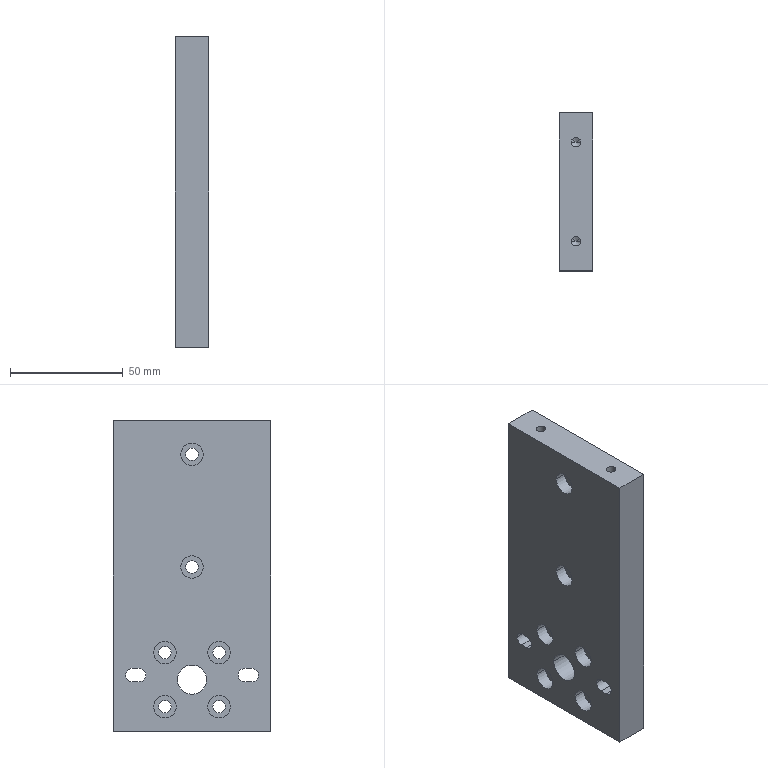Component | SolidWorks | OuterBagSealingSupportPlate-1 | 1 solid | 56 faces | box 15 x 70 x 138 mm | volume 137253 mm3 | cylinder 36 | plane 16 | cone 4 | commonest cylinder face diameters 10 x12 5.5 x12 6 x6 4.2 x4 13 x2
build123d program:
from build123d import *

# Parameters (mm, degrees)
SKETCH1_W                                       = 70
SKETCH1_H                                       = 138
SKETCH1_R                                       = 6.5
BOSS_EXTRUDE1_DEPTH                             = 7.5
M5_HEX_SOCKET_HEAD_CAP_SCREW_CBORE1_D           = 5.5
M5_HEX_SOCKET_HEAD_CAP_SCREW_CBORE1_CBORE_D     = 10
M5_HEX_SOCKET_HEAD_CAP_SCREW_CBORE1_CBORE_DEPTH = 5.4
M5_HEX_SOCKET_HEAD_CAP_SCREW_CBORE2_D           = 5.5
M5_HEX_SOCKET_HEAD_CAP_SCREW_CBORE2_CBORE_D     = 10
M5_HEX_SOCKET_HEAD_CAP_SCREW_CBORE2_CBORE_DEPTH = 5.4
CUT_EXTRUDE1_DEPTH                              = 15
M5_TAPPED_HOLE1_D                               = 4.2
M5_TAPPED_HOLE1_DEPTH                           = 12.4
M5_TAPPED_HOLE1_TIP                             = 1.212


with BuildPart() as part:
    # Sketch1 → Boss-Extrude1 (new, symmetric)
    with BuildSketch(Plane.XY):
        with Locations((35, 69)):
            Rectangle(SKETCH1_W, SKETCH1_H)
        with Locations((35, 115)):
            Circle(SKETCH1_R, mode=Mode.SUBTRACT)
    extrude(amount=BOSS_EXTRUDE1_DEPTH, both=True)

    # M5 Hex Socket Head Cap Screw CBORE1 (through all)
    with Locations(Plane(origin=(23, 127, 7.5), x_dir=(1, 0, 0), z_dir=(0, 0, 1))):
        with Locations((0, 0), (24, 0), (24, -24), (0, -24)):
            CounterBoreHole(M5_HEX_SOCKET_HEAD_CAP_SCREW_CBORE1_D / 2, M5_HEX_SOCKET_HEAD_CAP_SCREW_CBORE1_CBORE_D / 2, M5_HEX_SOCKET_HEAD_CAP_SCREW_CBORE1_CBORE_DEPTH)

    # M5 Hex Socket Head Cap Screw CBORE2 (through all)
    with Locations(Plane(origin=(35, 65, 7.5), x_dir=(1, 0, 0), z_dir=(0, 0, 1))):
        with Locations((0, 0), (0, -50)):
            CounterBoreHole(M5_HEX_SOCKET_HEAD_CAP_SCREW_CBORE2_D / 2, M5_HEX_SOCKET_HEAD_CAP_SCREW_CBORE2_CBORE_D / 2, M5_HEX_SOCKET_HEAD_CAP_SCREW_CBORE2_CBORE_DEPTH)

    # Sketch4 → Cut-Extrude1 (cut)
    with BuildSketch(Plane.XY.offset(7.5)):
        with BuildLine():
            Line((8.5, 116), (11.5, 116))
            ThreePointArc((11.5, 116), (14.5, 113), (11.5, 110))
            Line((11.5, 110), (8.5, 110))
            ThreePointArc((8.5, 110), (5.5, 113), (8.5, 116))
        make_face()
        with BuildLine():
            Line((58.5, 116), (61.5, 116))
            ThreePointArc((61.5, 116), (64.5, 113), (61.5, 110))
            Line((61.5, 110), (58.5, 110))
            ThreePointArc((58.5, 110), (55.5, 113), (58.5, 116))
        make_face()
    extrude(amount=-CUT_EXTRUDE1_DEPTH, mode=Mode.SUBTRACT)

    # M5 Tapped Hole1
    with Locations(Plane(origin=(13, 0, 0), x_dir=(0, 0, -1), z_dir=(0, -1, 0))):
        with Locations((0, 0), (0, 44)):
            Hole(M5_TAPPED_HOLE1_D / 2, depth=M5_TAPPED_HOLE1_DEPTH)
            with Locations((0, 0, -(M5_TAPPED_HOLE1_DEPTH + M5_TAPPED_HOLE1_TIP / 2))):  # 120° drill point
                Cone(0, M5_TAPPED_HOLE1_D / 2, M5_TAPPED_HOLE1_TIP, mode=Mode.SUBTRACT)


solid = part.part

# Placed as in the assembly
solid = solid.moved(Location((-4.585, 2.185, 71.225), (-90, -90, 0)))